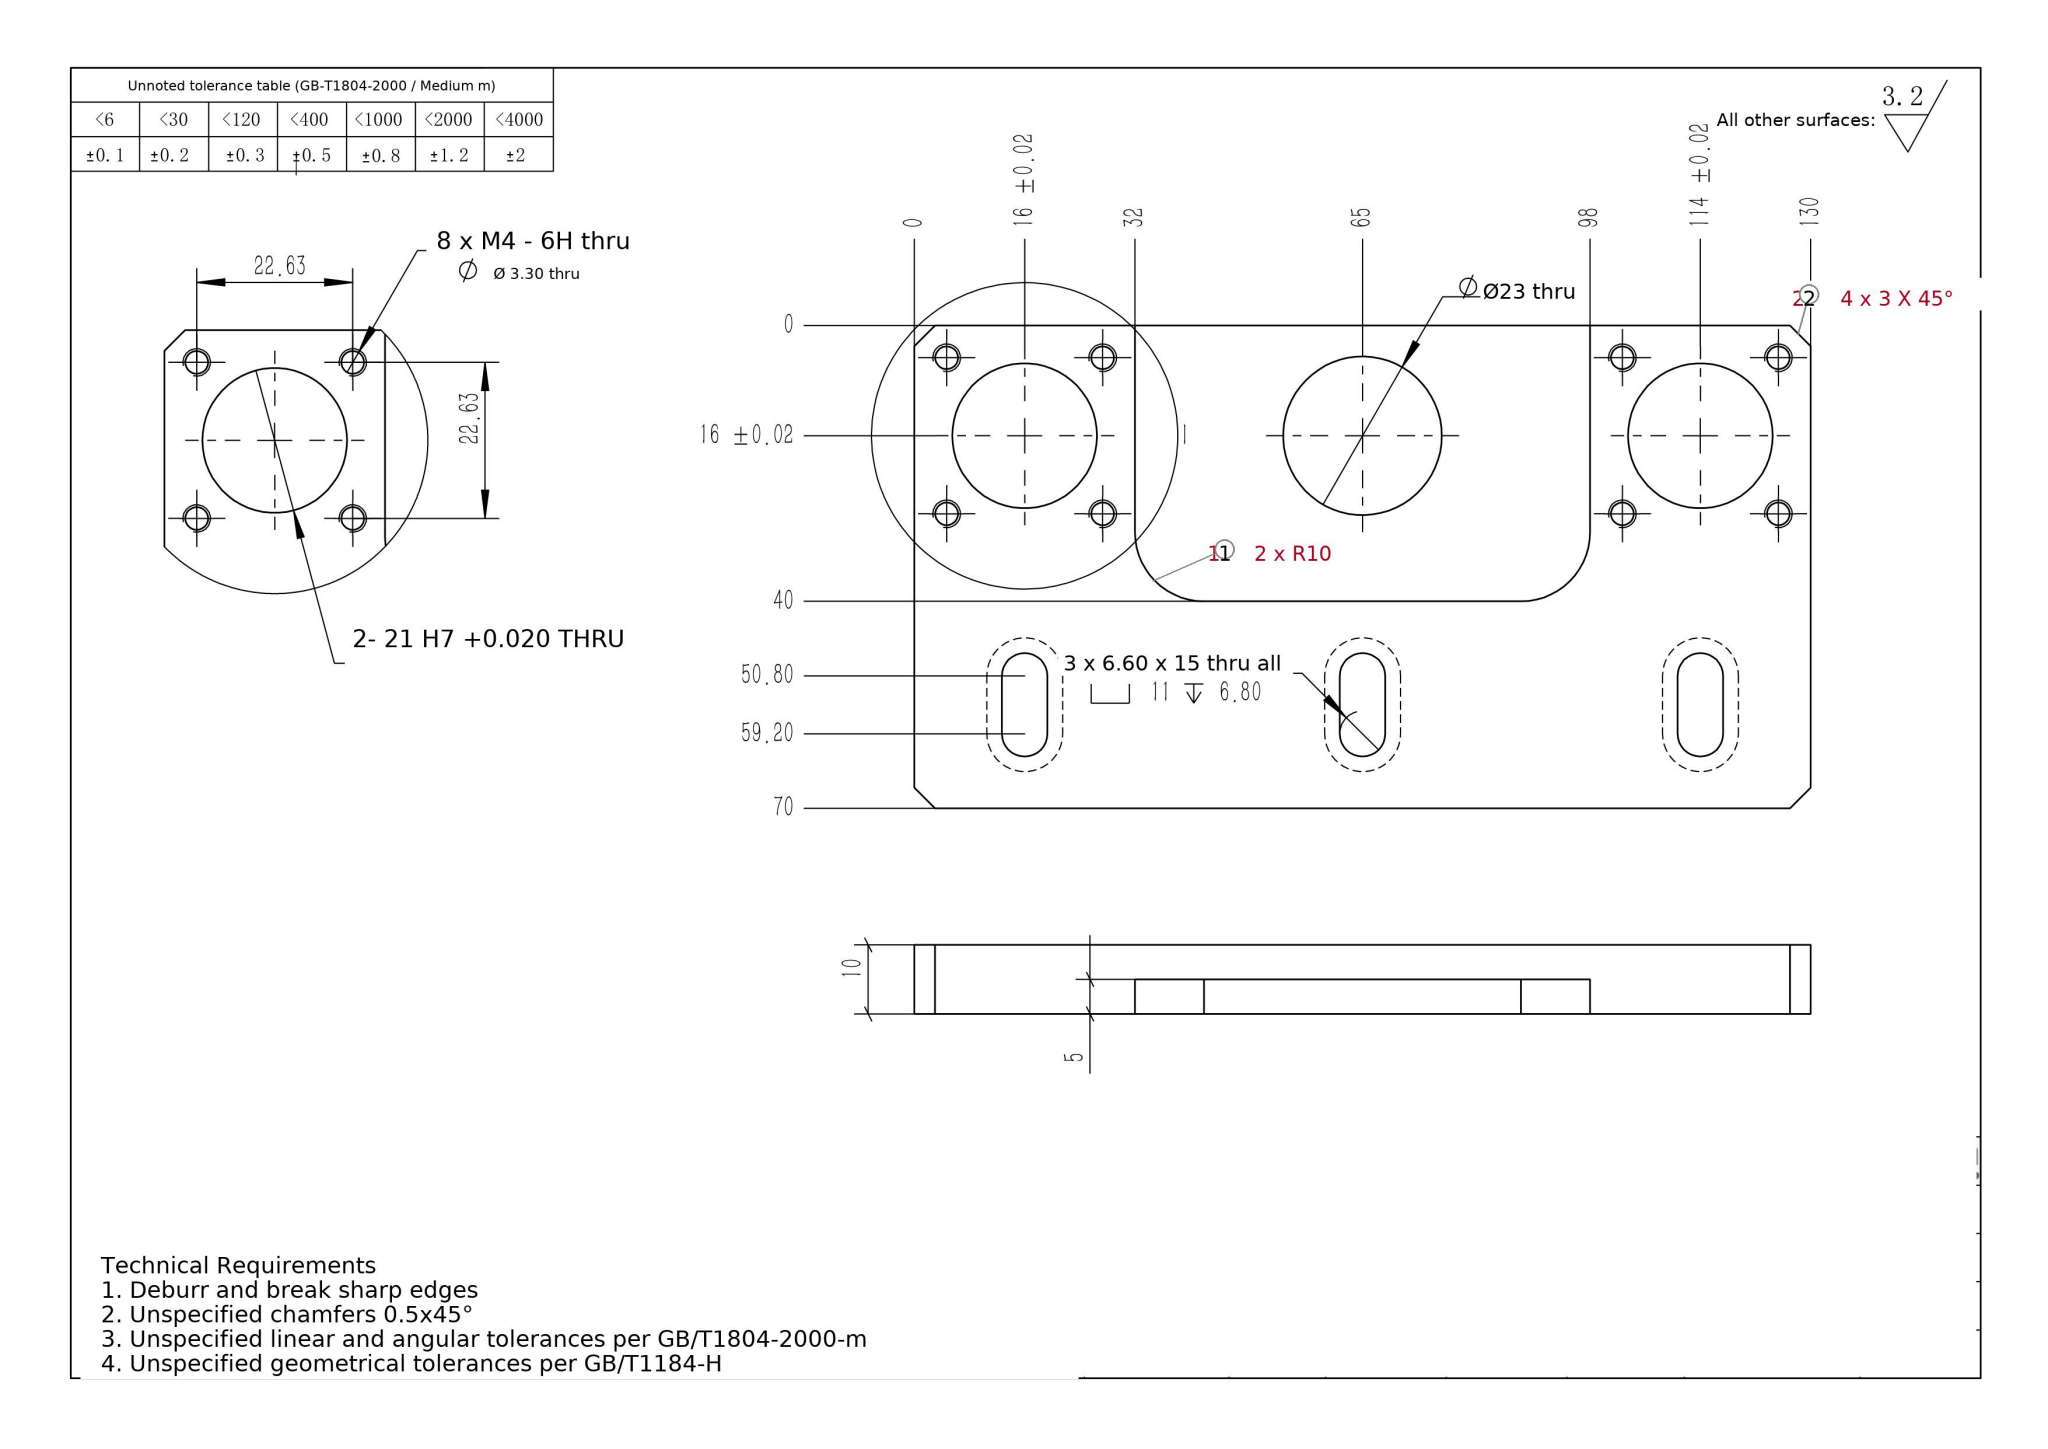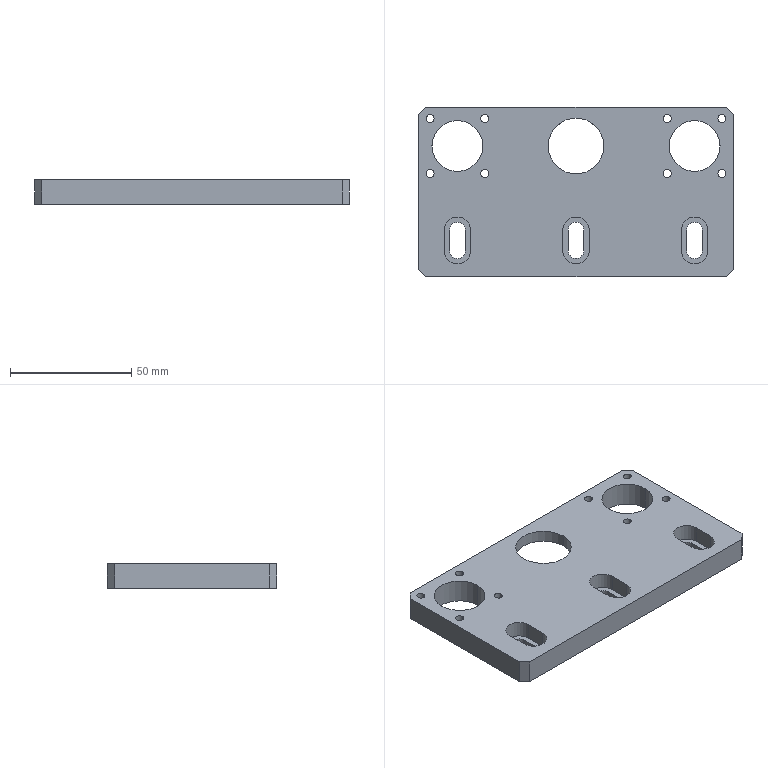Part | SolidWorks | mm | 1 solid | 65 faces | box 130 x 70 x 10 mm | volume 63461 mm3 | cylinder 36 | plane 29 | commonest cylinder face diameters 3.3 x16 6.6 x6 11 x6 21 x4 23 x2 20 x2